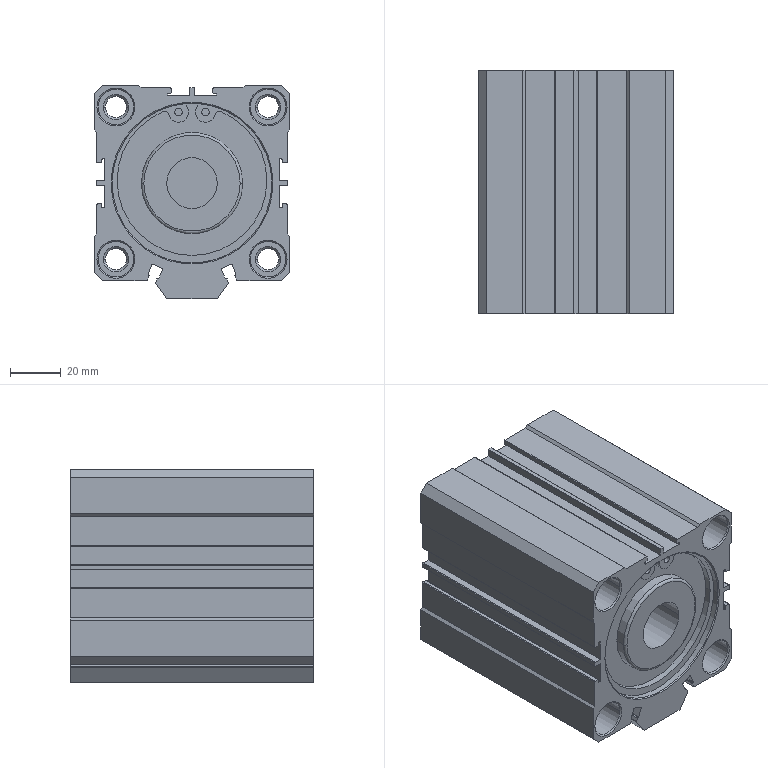Component | SolidWorks | ACQS_63x50_G_2_50-1_ACQS_63x5050_b-1 | 1 solid | 246 faces | volume 270939 mm3 | cylinder 108 | plane 92 | cone 44 | torus 2 | commonest cylinder face diameters 0.4 x35 14 x16 0.8 x15 8.376 x8 63 x6 3 x6 2 x4 11.445 x4